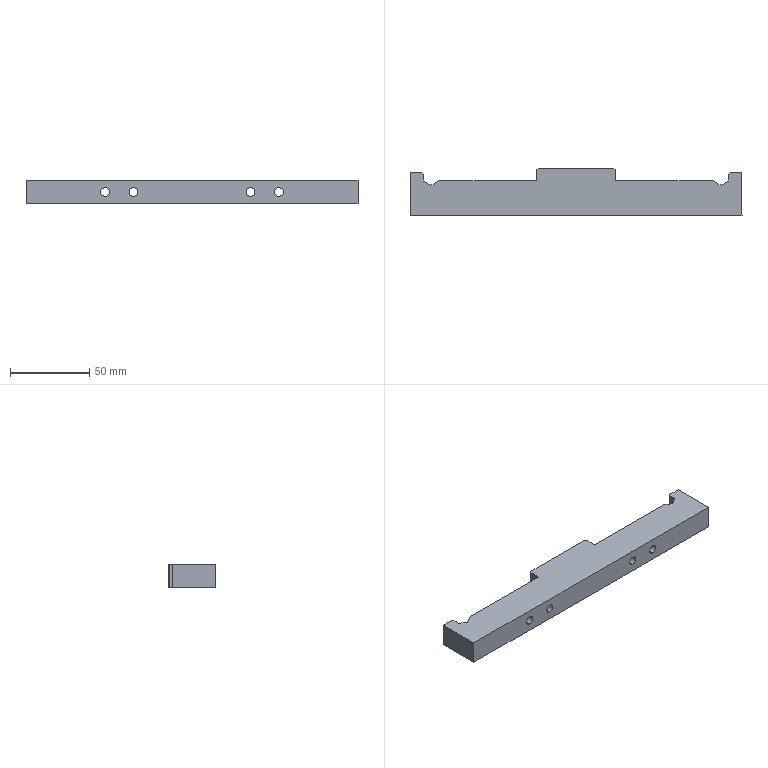Component | SolidWorks | YS01-072NozzleFasteningClampBlock2-1 | 1 solid | 46 faces | box 210 x 30.01 x 15 mm | volume 70004 mm3 | plane 22 | cylinder 16 | cone 8 | commonest cylinder face diameters 5.5 x8 11.2 x8
build123d program:
from build123d import *

# Parameters (mm, degrees)
SKETCH2_W                                            = 210
SKETCH2_H                                            = 30
BOSS_EXTRUDE1_DEPTH                                  = 15
CUT_EXTRUDE1_DEPTH                                   = 131.761
CHAMFER2_SIZE                                        = 1
SKETCH7_R                                            = 5.6
CUT_EXTRUDE3_DEPTH                                   = 12
M5_HEX_SOCKET_COUNTERSUNK_HEAD_SCREW_COU_D           = 5.5
M5_HEX_SOCKET_COUNTERSUNK_HEAD_SCREW_COU_CSINK_D     = 11.2
M5_HEX_SOCKET_COUNTERSUNK_HEAD_SCREW_COU_CSINK_ANGLE = 90


with BuildPart() as part:
    # Sketch2 → Boss-Extrude1 (new body)
    with BuildSketch(Plane.XY):
        with Locations((22.5, -9.842)):
            Rectangle(SKETCH2_W, SKETCH2_H)
    extrude(amount=-BOSS_EXTRUDE1_DEPTH)

    # Sketch3 → Cut-Extrude1 (cut, through all)
    with BuildSketch(Plane.XY):
        Polygon((-64.35, -2.891), (-2.45, -2.891), (-2.45, 6.586), (47.45, 6.586), (47.45, -2.891), (109.35, -2.891), (114.3, -5.749), (119.15, -2.949), (119.15, 2.458), (174.624, 2.458), (174.624, 20.896), (-96.14, 20.896), (-96.14, 2.458), (-74.15, 2.458), (-74.15, -2.949), (-69.3, -5.749), align=None)
    extrude(amount=-CUT_EXTRUDE1_DEPTH, mode=Mode.SUBTRACT)

    # Chamfer2
    chamfer2_edges = [part.edges().sort_by_distance(p)[0] for p in [
        (-2.45, 5.158, -7.5),
        (47.45, 5.158, -7.5),
        (-74.15, 2.458, -7.5),
        (119.15, 2.458, -7.5),
    ]]
    chamfer(chamfer2_edges, length=CHAMFER2_SIZE)

    # Sketch7 → Cut-Extrude3 (cut)
    with BuildSketch(Plane(origin=(0, -2.891, 0), x_dir=(1, 0, 0), z_dir=(0, 1, 0))):
        with Locations(Location((-32.5, 7.477, 0), (0, 0, 270))):
            Circle(SKETCH7_R)
        with Locations(Location((-14.5, 7.477, 0), (0, 0, 270))):
            Circle(SKETCH7_R)
    cut_extrude3 = extrude(amount=-CUT_EXTRUDE3_DEPTH, mode=Mode.SUBTRACT)

    # M5 Hex Socket Countersunk Head Screw Cou (through all)
    with Locations(Plane(origin=(0, -14.891, 0), x_dir=(1, 0, 0), z_dir=(0, 1, 0))):
        with Locations((-32.5, 7.477), (-14.5, 7.477)):
            m5_hex_socket_countersunk_head_screw_cou = CounterSinkHole(M5_HEX_SOCKET_COUNTERSUNK_HEAD_SCREW_COU_D / 2, M5_HEX_SOCKET_COUNTERSUNK_HEAD_SCREW_COU_CSINK_D / 2, counter_sink_angle=M5_HEX_SOCKET_COUNTERSUNK_HEAD_SCREW_COU_CSINK_ANGLE)

    # Mirror1: Cut-Extrude3, M5 Hex Socket Countersunk Head Screw Cou across plane
    add(cut_extrude3.mirror(Plane(origin=(22.5, 0, 0), x_dir=(0, 0, 1), z_dir=(1, 0, 0))), mode=Mode.SUBTRACT)
    add(m5_hex_socket_countersunk_head_screw_cou.mirror(Plane(origin=(22.5, 0, 0), x_dir=(0, 0, 1), z_dir=(1, 0, 0))), mode=Mode.SUBTRACT)


solid = part.part

# Placed as in the assembly
solid = solid.moved(Location((-589.111, -348.135, 2414.877), (0, 0, 0)))